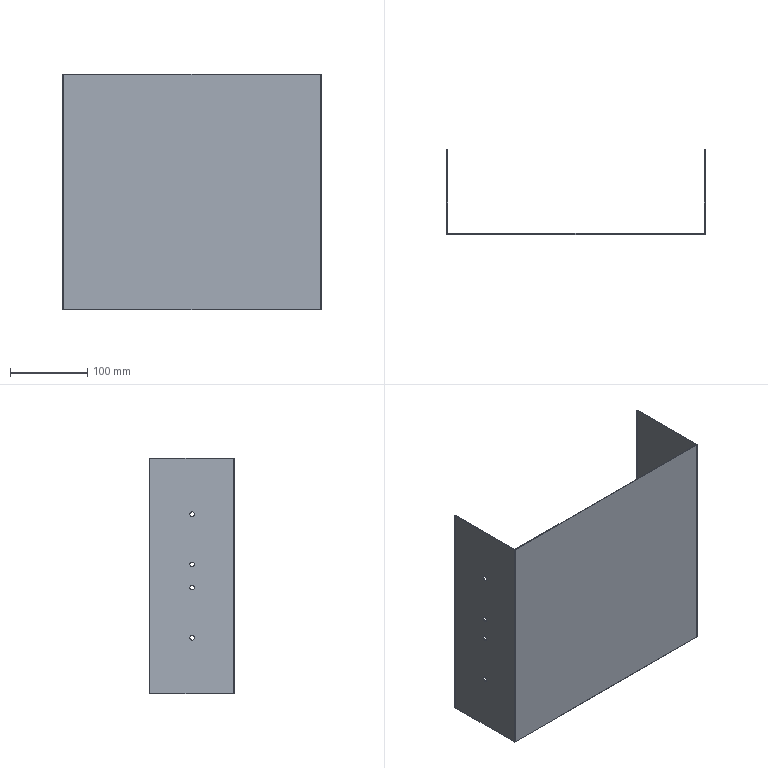Component | SolidWorks | WeldmentDrawing-1_DrawerBox-1 | 1 solid | 38 faces | box 335 x 110 x 305 mm | volume 168282 mm3 | cylinder 20 | plane 18 | commonest cylinder face diameters 6 x16 2.2 x2 0.2 x2
STEP:
#1=COLOUR_RGB('',0.7922,0.8196,0.9333);
#2=FILL_AREA_STYLE_COLOUR('',#1);
#3=FILL_AREA_STYLE('',(#2));
#4=SURFACE_STYLE_FILL_AREA(#3);
#5=SURFACE_SIDE_STYLE('',(#4));
#6=SURFACE_STYLE_USAGE(.BOTH.,#5);
#7=PRESENTATION_STYLE_ASSIGNMENT((#6));
#8=CARTESIAN_POINT('',(-7.849,-9.742,-0.09842));
#9=VERTEX_POINT('',#8);
#10=CARTESIAN_POINT('',(-7.849,-9.506,-0.09842));
#11=VERTEX_POINT('',#10);
#12=CARTESIAN_POINT('',(-7.849,-9.624,-0.09842));
#13=DIRECTION('',(1.,-0.,0.));
#14=DIRECTION('',(0.,-1.,0.));
#15=AXIS2_PLACEMENT_3D('',#12,#13,#14);
#16=CIRCLE('',#15,0.1181);
#17=EDGE_CURVE('',#9,#11,#16,.T.);
#18=ORIENTED_EDGE('',*,*,#17,.F.);
#19=CARTESIAN_POINT('',(-7.809,-9.742,-0.09842));
#20=VERTEX_POINT('',#19);
#21=CARTESIAN_POINT('',(-7.849,-9.742,-0.09842));
#22=DIRECTION('',(1.,-0.,0.));
#23=VECTOR('',#22,39.37);
#24=LINE('',#21,#23);
#25=EDGE_CURVE('',#9,#20,#24,.T.);
#26=ORIENTED_EDGE('',*,*,#25,.T.);
#27=CARTESIAN_POINT('',(-7.809,-9.506,-0.09842));
#28=VERTEX_POINT('',#27);
#29=CARTESIAN_POINT('',(-7.809,-9.624,-0.09842));
#30=DIRECTION('',(1.,0.,0.));
#31=DIRECTION('',(0.,1.,0.));
#32=AXIS2_PLACEMENT_3D('',#29,#30,#31);
#33=CIRCLE('',#32,0.1181);
#34=EDGE_CURVE('',#20,#28,#33,.T.);
#35=ORIENTED_EDGE('',*,*,#34,.T.);
#36=CARTESIAN_POINT('',(-7.849,-9.506,-0.09842));
#37=DIRECTION('',(1.,-0.,0.));
#38=VECTOR('',#37,39.37);
#39=LINE('',#36,#38);
#40=EDGE_CURVE('',#11,#28,#39,.T.);
#41=ORIENTED_EDGE('',*,*,#40,.F.);
#42=EDGE_LOOP('',(#18,#26,#35,#41));
#43=FACE_OUTER_BOUND('',#42,.T.);
#44=CARTESIAN_POINT('',(-7.849,-9.624,-0.09842));
#45=DIRECTION('',(1.,-0.,0.));
#46=DIRECTION('',(0.,1.,0.));
#47=AXIS2_PLACEMENT_3D('',#44,#45,#46);
#48=CYLINDRICAL_SURFACE('',#47,0.1181);
#49=ADVANCED_FACE('',(#43),#48,.F.);
#50=CARTESIAN_POINT('',(5.301,-9.506,-0.09842));
#51=VERTEX_POINT('',#50);
#52=CARTESIAN_POINT('',(5.301,-9.742,-0.09842));
#53=VERTEX_POINT('',#52);
#54=CARTESIAN_POINT('',(5.301,-9.624,-0.09842));
#55=DIRECTION('',(-1.,0.,0.));
#56=DIRECTION('',(0.,-1.,0.));
#57=AXIS2_PLACEMENT_3D('',#54,#55,#56);
#58=CIRCLE('',#57,0.1181);
#59=EDGE_CURVE('',#51,#53,#58,.T.);
#60=ORIENTED_EDGE('',*,*,#59,.T.);
#61=CARTESIAN_POINT('',(5.34,-9.742,-0.09842));
#62=VERTEX_POINT('',#61);
#63=CARTESIAN_POINT('',(-7.849,-9.742,-0.09842));
#64=DIRECTION('',(1.,-0.,0.));
#65=VECTOR('',#64,39.37);
#66=LINE('',#63,#65);
#67=EDGE_CURVE('',#53,#62,#66,.T.);
#68=ORIENTED_EDGE('',*,*,#67,.T.);
#69=CARTESIAN_POINT('',(5.34,-9.506,-0.09842));
#70=VERTEX_POINT('',#69);
#71=CARTESIAN_POINT('',(5.34,-9.624,-0.09842));
#72=DIRECTION('',(1.,-0.,0.));
#73=DIRECTION('',(0.,-1.,0.));
#74=AXIS2_PLACEMENT_3D('',#71,#72,#73);
#75=CIRCLE('',#74,0.1181);
#76=EDGE_CURVE('',#62,#70,#75,.T.);
#77=ORIENTED_EDGE('',*,*,#76,.T.);
#78=CARTESIAN_POINT('',(-7.849,-9.506,-0.09842));
#79=DIRECTION('',(1.,-0.,0.));
#80=VECTOR('',#79,39.37);
#81=LINE('',#78,#80);
#82=EDGE_CURVE('',#51,#70,#81,.T.);
#83=ORIENTED_EDGE('',*,*,#82,.F.);
#84=EDGE_LOOP('',(#60,#68,#77,#83));
#85=FACE_OUTER_BOUND('',#84,.T.);
#86=CARTESIAN_POINT('',(-7.849,-9.624,-0.09842));
#87=DIRECTION('',(1.,-0.,0.));
#88=DIRECTION('',(0.,1.,0.));
#89=AXIS2_PLACEMENT_3D('',#86,#87,#88);
#90=CYLINDRICAL_SURFACE('',#89,0.1181);
#91=ADVANCED_FACE('',(#85),#90,.F.);
#92=CARTESIAN_POINT('',(-7.849,-9.742,2.461));
#93=VERTEX_POINT('',#92);
#94=CARTESIAN_POINT('',(-7.849,-9.506,2.461));
#95=VERTEX_POINT('',#94);
#96=CARTESIAN_POINT('',(-7.849,-9.624,2.461));
#97=DIRECTION('',(1.,-0.,0.));
#98=DIRECTION('',(0.,-1.,0.));
#99=AXIS2_PLACEMENT_3D('',#96,#97,#98);
#100=CIRCLE('',#99,0.1181);
#101=EDGE_CURVE('',#93,#95,#100,.T.);
#102=ORIENTED_EDGE('',*,*,#101,.F.);
#103=CARTESIAN_POINT('',(-7.809,-9.742,2.461));
#104=VERTEX_POINT('',#103);
#105=CARTESIAN_POINT('',(-7.849,-9.742,2.461));
#106=DIRECTION('',(1.,-0.,0.));
#107=VECTOR('',#106,39.37);
#108=LINE('',#105,#107);
#109=EDGE_CURVE('',#93,#104,#108,.T.);
#110=ORIENTED_EDGE('',*,*,#109,.T.);
#111=CARTESIAN_POINT('',(-7.809,-9.506,2.461));
#112=VERTEX_POINT('',#111);
#113=CARTESIAN_POINT('',(-7.809,-9.624,2.461));
#114=DIRECTION('',(1.,0.,0.));
#115=DIRECTION('',(0.,1.,0.));
#116=AXIS2_PLACEMENT_3D('',#113,#114,#115);
#117=CIRCLE('',#116,0.1181);
#118=EDGE_CURVE('',#104,#112,#117,.T.);
#119=ORIENTED_EDGE('',*,*,#118,.T.);
#120=CARTESIAN_POINT('',(-7.849,-9.506,2.461));
#121=DIRECTION('',(1.,-0.,0.));
#122=VECTOR('',#121,39.37);
#123=LINE('',#120,#122);
#124=EDGE_CURVE('',#95,#112,#123,.T.);
#125=ORIENTED_EDGE('',*,*,#124,.F.);
#126=EDGE_LOOP('',(#102,#110,#119,#125));
#127=FACE_OUTER_BOUND('',#126,.T.);
#128=CARTESIAN_POINT('',(-7.849,-9.624,2.461));
#129=DIRECTION('',(1.,-0.,0.));
#130=DIRECTION('',(0.,1.,0.));
#131=AXIS2_PLACEMENT_3D('',#128,#129,#130);
#132=CYLINDRICAL_SURFACE('',#131,0.1181);
#133=ADVANCED_FACE('',(#127),#132,.F.);
#134=CARTESIAN_POINT('',(5.301,-9.506,2.461));
#135=VERTEX_POINT('',#134);
#136=CARTESIAN_POINT('',(5.301,-9.742,2.461));
#137=VERTEX_POINT('',#136);
#138=CARTESIAN_POINT('',(5.301,-9.624,2.461));
#139=DIRECTION('',(-1.,0.,0.));
#140=DIRECTION('',(0.,-1.,0.));
#141=AXIS2_PLACEMENT_3D('',#138,#139,#140);
#142=CIRCLE('',#141,0.1181);
#143=EDGE_CURVE('',#135,#137,#142,.T.);
#144=ORIENTED_EDGE('',*,*,#143,.T.);
#145=CARTESIAN_POINT('',(5.34,-9.742,2.461));
#146=VERTEX_POINT('',#145);
#147=CARTESIAN_POINT('',(-7.849,-9.742,2.461));
#148=DIRECTION('',(1.,-0.,0.));
#149=VECTOR('',#148,39.37);
#150=LINE('',#147,#149);
#151=EDGE_CURVE('',#137,#146,#150,.T.);
#152=ORIENTED_EDGE('',*,*,#151,.T.);
#153=CARTESIAN_POINT('',(5.34,-9.506,2.461));
#154=VERTEX_POINT('',#153);
#155=CARTESIAN_POINT('',(5.34,-9.624,2.461));
#156=DIRECTION('',(1.,-0.,0.));
#157=DIRECTION('',(0.,-1.,0.));
#158=AXIS2_PLACEMENT_3D('',#155,#156,#157);
#159=CIRCLE('',#158,0.1181);
#160=EDGE_CURVE('',#146,#154,#159,.T.);
#161=ORIENTED_EDGE('',*,*,#160,.T.);
#162=CARTESIAN_POINT('',(-7.849,-9.506,2.461));
#163=DIRECTION('',(1.,-0.,0.));
#164=VECTOR('',#163,39.37);
#165=LINE('',#162,#164);
#166=EDGE_CURVE('',#135,#154,#165,.T.);
#167=ORIENTED_EDGE('',*,*,#166,.F.);
#168=EDGE_LOOP('',(#144,#152,#161,#167));
#169=FACE_OUTER_BOUND('',#168,.T.);
#170=CARTESIAN_POINT('',(-7.849,-9.624,2.461));
#171=DIRECTION('',(1.,-0.,0.));
#172=DIRECTION('',(0.,1.,0.));
#173=AXIS2_PLACEMENT_3D('',#170,#171,#172);
#174=CYLINDRICAL_SURFACE('',#173,0.1181);
#175=ADVANCED_FACE('',(#169),#174,.F.);
#176=CARTESIAN_POINT('',(-7.849,-9.742,3.642));
#177=VERTEX_POINT('',#176);
#178=CARTESIAN_POINT('',(-7.849,-9.506,3.642));
#179=VERTEX_POINT('',#178);
#180=CARTESIAN_POINT('',(-7.849,-9.624,3.642));
#181=DIRECTION('',(1.,-0.,0.));
#182=DIRECTION('',(0.,1.,0.));
#183=AXIS2_PLACEMENT_3D('',#180,#181,#182);
#184=CIRCLE('',#183,0.1181);
#185=EDGE_CURVE('',#177,#179,#184,.T.);
#186=ORIENTED_EDGE('',*,*,#185,.F.);
#187=CARTESIAN_POINT('',(-7.809,-9.742,3.642));
#188=VERTEX_POINT('',#187);
#189=CARTESIAN_POINT('',(-7.849,-9.742,3.642));
#190=DIRECTION('',(1.,-0.,0.));
#191=VECTOR('',#190,39.37);
#192=LINE('',#189,#191);
#193=EDGE_CURVE('',#177,#188,#192,.T.);
#194=ORIENTED_EDGE('',*,*,#193,.T.);
#195=CARTESIAN_POINT('',(-7.809,-9.506,3.642));
#196=VERTEX_POINT('',#195);
#197=CARTESIAN_POINT('',(-7.809,-9.624,3.642));
#198=DIRECTION('',(1.,0.,0.));
#199=DIRECTION('',(0.,1.,0.));
#200=AXIS2_PLACEMENT_3D('',#197,#198,#199);
#201=CIRCLE('',#200,0.1181);
#202=EDGE_CURVE('',#188,#196,#201,.T.);
#203=ORIENTED_EDGE('',*,*,#202,.T.);
#204=CARTESIAN_POINT('',(-7.849,-9.506,3.642));
#205=DIRECTION('',(1.,-0.,0.));
#206=VECTOR('',#205,39.37);
#207=LINE('',#204,#206);
#208=EDGE_CURVE('',#179,#196,#207,.T.);
#209=ORIENTED_EDGE('',*,*,#208,.F.);
#210=EDGE_LOOP('',(#186,#194,#203,#209));
#211=FACE_OUTER_BOUND('',#210,.T.);
#212=CARTESIAN_POINT('',(-7.849,-9.624,3.642));
#213=DIRECTION('',(1.,-0.,0.));
#214=DIRECTION('',(0.,1.,0.));
#215=AXIS2_PLACEMENT_3D('',#212,#213,#214);
#216=CYLINDRICAL_SURFACE('',#215,0.1181);
#217=ADVANCED_FACE('',(#211),#216,.F.);
#218=CARTESIAN_POINT('',(5.301,-9.506,3.642));
#219=VERTEX_POINT('',#218);
#220=CARTESIAN_POINT('',(5.301,-9.742,3.642));
#221=VERTEX_POINT('',#220);
#222=CARTESIAN_POINT('',(5.301,-9.624,3.642));
#223=DIRECTION('',(-1.,0.,0.));
#224=DIRECTION('',(0.,-1.,0.));
#225=AXIS2_PLACEMENT_3D('',#222,#223,#224);
#226=CIRCLE('',#225,0.1181);
#227=EDGE_CURVE('',#219,#221,#226,.T.);
#228=ORIENTED_EDGE('',*,*,#227,.T.);
#229=CARTESIAN_POINT('',(5.34,-9.742,3.642));
#230=VERTEX_POINT('',#229);
#231=CARTESIAN_POINT('',(-7.849,-9.742,3.642));
#232=DIRECTION('',(1.,-0.,0.));
#233=VECTOR('',#232,39.37);
#234=LINE('',#231,#233);
#235=EDGE_CURVE('',#221,#230,#234,.T.);
#236=ORIENTED_EDGE('',*,*,#235,.T.);
#237=CARTESIAN_POINT('',(5.34,-9.506,3.642));
#238=VERTEX_POINT('',#237);
#239=CARTESIAN_POINT('',(5.34,-9.624,3.642));
#240=DIRECTION('',(1.,-0.,0.));
#241=DIRECTION('',(0.,1.,0.));
#242=AXIS2_PLACEMENT_3D('',#239,#240,#241);
#243=CIRCLE('',#242,0.1181);
#244=EDGE_CURVE('',#230,#238,#243,.T.);
#245=ORIENTED_EDGE('',*,*,#244,.T.);
#246=CARTESIAN_POINT('',(-7.849,-9.506,3.642));
#247=DIRECTION('',(1.,-0.,0.));
#248=VECTOR('',#247,39.37);
#249=LINE('',#246,#248);
#250=EDGE_CURVE('',#219,#238,#249,.T.);
#251=ORIENTED_EDGE('',*,*,#250,.F.);
#252=EDGE_LOOP('',(#228,#236,#245,#251));
#253=FACE_OUTER_BOUND('',#252,.T.);
#254=CARTESIAN_POINT('',(-7.849,-9.624,3.642));
#255=DIRECTION('',(1.,-0.,0.));
#256=DIRECTION('',(0.,1.,0.));
#257=AXIS2_PLACEMENT_3D('',#254,#255,#256);
#258=CYLINDRICAL_SURFACE('',#257,0.1181);
#259=ADVANCED_FACE('',(#253),#258,.F.);
#260=CARTESIAN_POINT('',(-7.849,-9.742,6.201));
#261=VERTEX_POINT('',#260);
#262=CARTESIAN_POINT('',(-7.849,-9.506,6.201));
#263=VERTEX_POINT('',#262);
#264=CARTESIAN_POINT('',(-7.849,-9.624,6.201));
#265=DIRECTION('',(1.,-0.,0.));
#266=DIRECTION('',(0.,1.,0.));
#267=AXIS2_PLACEMENT_3D('',#264,#265,#266);
#268=CIRCLE('',#267,0.1181);
#269=EDGE_CURVE('',#261,#263,#268,.T.);
#270=ORIENTED_EDGE('',*,*,#269,.F.);
#271=CARTESIAN_POINT('',(-7.809,-9.742,6.201));
#272=VERTEX_POINT('',#271);
#273=CARTESIAN_POINT('',(-7.849,-9.742,6.201));
#274=DIRECTION('',(1.,-0.,0.));
#275=VECTOR('',#274,39.37);
#276=LINE('',#273,#275);
#277=EDGE_CURVE('',#261,#272,#276,.T.);
#278=ORIENTED_EDGE('',*,*,#277,.T.);
#279=CARTESIAN_POINT('',(-7.809,-9.506,6.201));
#280=VERTEX_POINT('',#279);
#281=CARTESIAN_POINT('',(-7.809,-9.624,6.201));
#282=DIRECTION('',(1.,0.,0.));
#283=DIRECTION('',(0.,1.,0.));
#284=AXIS2_PLACEMENT_3D('',#281,#282,#283);
#285=CIRCLE('',#284,0.1181);
#286=EDGE_CURVE('',#272,#280,#285,.T.);
#287=ORIENTED_EDGE('',*,*,#286,.T.);
#288=CARTESIAN_POINT('',(-7.849,-9.506,6.201));
#289=DIRECTION('',(1.,-0.,0.));
#290=VECTOR('',#289,39.37);
#291=LINE('',#288,#290);
#292=EDGE_CURVE('',#263,#280,#291,.T.);
#293=ORIENTED_EDGE('',*,*,#292,.F.);
#294=EDGE_LOOP('',(#270,#278,#287,#293));
#295=FACE_OUTER_BOUND('',#294,.T.);
#296=CARTESIAN_POINT('',(-7.849,-9.624,6.201));
#297=DIRECTION('',(1.,-0.,0.));
#298=DIRECTION('',(0.,1.,0.));
#299=AXIS2_PLACEMENT_3D('',#296,#297,#298);
#300=CYLINDRICAL_SURFACE('',#299,0.1181);
#301=ADVANCED_FACE('',(#295),#300,.F.);
#302=CARTESIAN_POINT('',(5.301,-9.506,6.201));
#303=VERTEX_POINT('',#302);
#304=CARTESIAN_POINT('',(5.301,-9.742,6.201));
#305=VERTEX_POINT('',#304);
#306=CARTESIAN_POINT('',(5.301,-9.624,6.201));
#307=DIRECTION('',(-1.,0.,0.));
#308=DIRECTION('',(0.,-1.,0.));
#309=AXIS2_PLACEMENT_3D('',#306,#307,#308);
#310=CIRCLE('',#309,0.1181);
#311=EDGE_CURVE('',#303,#305,#310,.T.);
#312=ORIENTED_EDGE('',*,*,#311,.T.);
#313=CARTESIAN_POINT('',(5.34,-9.742,6.201));
#314=VERTEX_POINT('',#313);
#315=CARTESIAN_POINT('',(-7.849,-9.742,6.201));
#316=DIRECTION('',(1.,-0.,0.));
#317=VECTOR('',#316,39.37);
#318=LINE('',#315,#317);
#319=EDGE_CURVE('',#305,#314,#318,.T.);
#320=ORIENTED_EDGE('',*,*,#319,.T.);
#321=CARTESIAN_POINT('',(5.34,-9.506,6.201));
#322=VERTEX_POINT('',#321);
#323=CARTESIAN_POINT('',(5.34,-9.624,6.201));
#324=DIRECTION('',(1.,-0.,0.));
#325=DIRECTION('',(0.,1.,0.));
#326=AXIS2_PLACEMENT_3D('',#323,#324,#325);
#327=CIRCLE('',#326,0.1181);
#328=EDGE_CURVE('',#314,#322,#327,.T.);
#329=ORIENTED_EDGE('',*,*,#328,.T.);
#330=CARTESIAN_POINT('',(-7.849,-9.506,6.201));
#331=DIRECTION('',(1.,-0.,0.));
#332=VECTOR('',#331,39.37);
#333=LINE('',#330,#332);
#334=EDGE_CURVE('',#303,#322,#333,.T.);
#335=ORIENTED_EDGE('',*,*,#334,.F.);
#336=EDGE_LOOP('',(#312,#320,#329,#335));
#337=FACE_OUTER_BOUND('',#336,.T.);
#338=CARTESIAN_POINT('',(-7.849,-9.624,6.201));
#339=DIRECTION('',(1.,-0.,0.));
#340=DIRECTION('',(0.,1.,0.));
#341=AXIS2_PLACEMENT_3D('',#338,#339,#340);
#342=CYLINDRICAL_SURFACE('',#341,0.1181);
#343=ADVANCED_FACE('',(#337),#342,.F.);
#344=CARTESIAN_POINT('',(5.297,-11.778,-2.953));
#345=VERTEX_POINT('',#344);
#346=CARTESIAN_POINT('',(-7.806,-11.778,-2.953));
#347=VERTEX_POINT('',#346);
#348=CARTESIAN_POINT('',(-7.849,-11.778,-2.953));
#349=DIRECTION('',(-1.,0.,0.));
#350=VECTOR('',#349,39.37);
#351=LINE('',#348,#350);
#352=EDGE_CURVE('',#345,#347,#351,.T.);
#353=ORIENTED_EDGE('',*,*,#352,.F.);
#354=CARTESIAN_POINT('',(5.297,-11.778,9.055));
#355=VERTEX_POINT('',#354);
#356=CARTESIAN_POINT('',(5.297,-11.778,-2.953));
#357=DIRECTION('',(0.,0.,1.));
#358=VECTOR('',#357,39.37);
#359=LINE('',#356,#358);
#360=EDGE_CURVE('',#345,#355,#359,.T.);
#361=ORIENTED_EDGE('',*,*,#360,.T.);
#362=CARTESIAN_POINT('',(-7.806,-11.778,9.055));
#363=VERTEX_POINT('',#362);
#364=CARTESIAN_POINT('',(-7.849,-11.778,9.055));
#365=DIRECTION('',(1.,0.,0.));
#366=VECTOR('',#365,39.37);
#367=LINE('',#364,#366);
#368=EDGE_CURVE('',#363,#355,#367,.T.);
#369=ORIENTED_EDGE('',*,*,#368,.F.);
#370=CARTESIAN_POINT('',(-7.806,-11.778,9.055));
#371=DIRECTION('',(0.,0.,-1.));
#372=VECTOR('',#371,39.37);
#373=LINE('',#370,#372);
#374=EDGE_CURVE('',#363,#347,#373,.T.);
#375=ORIENTED_EDGE('',*,*,#374,.T.);
#376=EDGE_LOOP('',(#353,#361,#369,#375));
#377=FACE_OUTER_BOUND('',#376,.T.);
#378=CARTESIAN_POINT('',(-5.646,-11.778,6.989));
#379=DIRECTION('',(0.,-1.,0.));
#380=DIRECTION('',(0.,0.,-1.));
#381=AXIS2_PLACEMENT_3D('',#378,#379,#380);
#382=PLANE('',#381);
#383=ADVANCED_FACE('',(#377),#382,.T.);
#384=CARTESIAN_POINT('',(5.297,-11.738,-2.953));
#385=VERTEX_POINT('',#384);
#386=CARTESIAN_POINT('',(5.297,-11.738,9.055));
#387=VERTEX_POINT('',#386);
#388=CARTESIAN_POINT('',(5.297,-11.738,-2.953));
#389=DIRECTION('',(0.,0.,1.));
#390=VECTOR('',#389,39.37);
#391=LINE('',#388,#390);
#392=EDGE_CURVE('',#385,#387,#391,.T.);
#393=ORIENTED_EDGE('',*,*,#392,.F.);
#394=CARTESIAN_POINT('',(-7.806,-11.738,-2.953));
#395=VERTEX_POINT('',#394);
#396=CARTESIAN_POINT('',(-7.849,-11.738,-2.953));
#397=DIRECTION('',(-1.,0.,0.));
#398=VECTOR('',#397,39.37);
#399=LINE('',#396,#398);
#400=EDGE_CURVE('',#385,#395,#399,.T.);
#401=ORIENTED_EDGE('',*,*,#400,.T.);
#402=CARTESIAN_POINT('',(-7.806,-11.738,9.055));
#403=VERTEX_POINT('',#402);
#404=CARTESIAN_POINT('',(-7.806,-11.738,9.055));
#405=DIRECTION('',(0.,0.,-1.));
#406=VECTOR('',#405,39.37);
#407=LINE('',#404,#406);
#408=EDGE_CURVE('',#403,#395,#407,.T.);
#409=ORIENTED_EDGE('',*,*,#408,.F.);
#410=CARTESIAN_POINT('',(-7.849,-11.738,9.055));
#411=DIRECTION('',(1.,0.,0.));
#412=VECTOR('',#411,39.37);
#413=LINE('',#410,#412);
#414=EDGE_CURVE('',#403,#387,#413,.T.);
#415=ORIENTED_EDGE('',*,*,#414,.T.);
#416=EDGE_LOOP('',(#393,#401,#409,#415));
#417=FACE_OUTER_BOUND('',#416,.T.);
#418=CARTESIAN_POINT('',(-5.646,-11.738,6.989));
#419=DIRECTION('',(0.,-1.,0.));
#420=DIRECTION('',(0.,0.,-1.));
#421=AXIS2_PLACEMENT_3D('',#418,#419,#420);
#422=PLANE('',#421);
#423=ADVANCED_FACE('',(#417),#422,.F.);
#424=ORIENTED_EDGE('',*,*,#400,.F.);
#425=CARTESIAN_POINT('',(5.297,-11.738,-2.953));
#426=DIRECTION('',(0.,-1.,-0.));
#427=VECTOR('',#426,39.37);
#428=LINE('',#425,#427);
#429=EDGE_CURVE('',#385,#345,#428,.T.);
#430=ORIENTED_EDGE('',*,*,#429,.T.);
#431=ORIENTED_EDGE('',*,*,#352,.T.);
#432=CARTESIAN_POINT('',(-7.806,-11.738,-2.953));
#433=DIRECTION('',(0.,-1.,0.));
#434=VECTOR('',#433,39.37);
#435=LINE('',#432,#434);
#436=EDGE_CURVE('',#395,#347,#435,.T.);
#437=ORIENTED_EDGE('',*,*,#436,.F.);
#438=EDGE_LOOP('',(#424,#430,#431,#437));
#439=FACE_OUTER_BOUND('',#438,.T.);
#440=CARTESIAN_POINT('',(-7.849,-11.778,-2.953));
#441=DIRECTION('',(0.,0.,-1.));
#442=DIRECTION('',(-1.,0.,0.));
#443=AXIS2_PLACEMENT_3D('',#440,#441,#442);
#444=PLANE('',#443);
#445=ADVANCED_FACE('',(#439),#444,.T.);
#446=CARTESIAN_POINT('',(5.297,-11.738,9.055));
#447=DIRECTION('',(0.,-1.,0.));
#448=VECTOR('',#447,39.37);
#449=LINE('',#446,#448);
#450=EDGE_CURVE('',#387,#355,#449,.T.);
#451=ORIENTED_EDGE('',*,*,#450,.F.);
#452=ORIENTED_EDGE('',*,*,#414,.F.);
#453=CARTESIAN_POINT('',(-7.806,-11.738,9.055));
#454=DIRECTION('',(0.,-1.,-0.));
#455=VECTOR('',#454,39.37);
#456=LINE('',#453,#455);
#457=EDGE_CURVE('',#403,#363,#456,.T.);
#458=ORIENTED_EDGE('',*,*,#457,.T.);
#459=ORIENTED_EDGE('',*,*,#368,.T.);
#460=EDGE_LOOP('',(#451,#452,#458,#459));
#461=FACE_OUTER_BOUND('',#460,.T.);
#462=CARTESIAN_POINT('',(-7.849,-11.778,9.055));
#463=DIRECTION('',(0.,0.,1.));
#464=DIRECTION('',(1.,0.,0.));
#465=AXIS2_PLACEMENT_3D('',#462,#463,#464);
#466=PLANE('',#465);
#467=ADVANCED_FACE('',(#461),#466,.T.);
#468=CARTESIAN_POINT('',(-7.809,-11.734,-2.953));
#469=VERTEX_POINT('',#468);
#470=CARTESIAN_POINT('',(-7.849,-11.734,-2.953));
#471=VERTEX_POINT('',#470);
#472=CARTESIAN_POINT('',(-7.849,-11.734,-2.953));
#473=DIRECTION('',(-1.,-0.,0.));
#474=VECTOR('',#473,39.37);
#475=LINE('',#472,#474);
#476=EDGE_CURVE('',#469,#471,#475,.T.);
#477=ORIENTED_EDGE('',*,*,#476,.F.);
#478=CARTESIAN_POINT('',(-7.806,-11.734,-2.953));
#479=DIRECTION('',(0.,0.,-1.));
#480=DIRECTION('',(0.,-1.,0.));
#481=AXIS2_PLACEMENT_3D('',#478,#479,#480);
#482=CIRCLE('',#481,0.003937);
#483=EDGE_CURVE('',#395,#469,#482,.T.);
#484=ORIENTED_EDGE('',*,*,#483,.F.);
#485=ORIENTED_EDGE('',*,*,#436,.T.);
#486=CARTESIAN_POINT('',(-7.806,-11.734,-2.953));
#487=DIRECTION('',(0.,0.,-1.));
#488=DIRECTION('',(0.,-1.,0.));
#489=AXIS2_PLACEMENT_3D('',#486,#487,#488);
#490=CIRCLE('',#489,0.04331);
#491=EDGE_CURVE('',#347,#471,#490,.T.);
#492=ORIENTED_EDGE('',*,*,#491,.T.);
#493=EDGE_LOOP('',(#477,#484,#485,#492));
#494=FACE_OUTER_BOUND('',#493,.T.);
#495=CARTESIAN_POINT('',(-7.806,-11.734,-2.953));
#496=DIRECTION('',(0.,0.,-1.));
#497=DIRECTION('',(0.,1.,0.));
#498=AXIS2_PLACEMENT_3D('',#495,#496,#497);
#499=PLANE('',#498);
#500=ADVANCED_FACE('',(#494),#499,.T.);
#501=CARTESIAN_POINT('',(-7.809,-11.734,9.055));
#502=VERTEX_POINT('',#501);
#503=CARTESIAN_POINT('',(-7.806,-11.734,9.055));
#504=DIRECTION('',(0.,-0.,1.));
#505=DIRECTION('',(0.,-1.,0.));
#506=AXIS2_PLACEMENT_3D('',#503,#504,#505);
#507=CIRCLE('',#506,0.003937);
#508=EDGE_CURVE('',#502,#403,#507,.T.);
#509=ORIENTED_EDGE('',*,*,#508,.F.);
#510=CARTESIAN_POINT('',(-7.849,-11.734,9.055));
#511=VERTEX_POINT('',#510);
#512=CARTESIAN_POINT('',(-7.809,-11.734,9.055));
#513=DIRECTION('',(-1.,-0.,0.));
#514=VECTOR('',#513,39.37);
#515=LINE('',#512,#514);
#516=EDGE_CURVE('',#502,#511,#515,.T.);
#517=ORIENTED_EDGE('',*,*,#516,.T.);
#518=CARTESIAN_POINT('',(-7.806,-11.734,9.055));
#519=DIRECTION('',(0.,-0.,1.));
#520=DIRECTION('',(0.,-1.,0.));
#521=AXIS2_PLACEMENT_3D('',#518,#519,#520);
#522=CIRCLE('',#521,0.04331);
#523=EDGE_CURVE('',#511,#363,#522,.T.);
#524=ORIENTED_EDGE('',*,*,#523,.T.);
#525=ORIENTED_EDGE('',*,*,#457,.F.);
#526=EDGE_LOOP('',(#509,#517,#524,#525));
#527=FACE_OUTER_BOUND('',#526,.T.);
#528=CARTESIAN_POINT('',(-7.806,-11.734,9.055));
#529=DIRECTION('',(0.,0.,-1.));
#530=DIRECTION('',(0.,1.,0.));
#531=AXIS2_PLACEMENT_3D('',#528,#529,#530);
#532=PLANE('',#531);
#533=ADVANCED_FACE('',(#527),#532,.F.);
#534=ORIENTED_EDGE('',*,*,#374,.F.);
#535=ORIENTED_EDGE('',*,*,#523,.F.);
#536=CARTESIAN_POINT('',(-7.849,-11.734,-2.953));
#537=DIRECTION('',(-0.,0.,-1.));
#538=VECTOR('',#537,39.37);
#539=LINE('',#536,#538);
#540=EDGE_CURVE('',#511,#471,#539,.T.);
#541=ORIENTED_EDGE('',*,*,#540,.T.);
#542=ORIENTED_EDGE('',*,*,#491,.F.);
#543=EDGE_LOOP('',(#534,#535,#541,#542));
#544=FACE_OUTER_BOUND('',#543,.T.);
#545=CARTESIAN_POINT('',(-7.806,-11.734,9.055));
#546=DIRECTION('',(0.,-0.,1.));
#547=DIRECTION('',(-1.,0.,0.));
#548=AXIS2_PLACEMENT_3D('',#545,#546,#547);
#549=CYLINDRICAL_SURFACE('',#548,0.04331);
#550=ADVANCED_FACE('',(#544),#549,.T.);
#551=ORIENTED_EDGE('',*,*,#408,.T.);
#552=ORIENTED_EDGE('',*,*,#483,.T.);
#553=CARTESIAN_POINT('',(-7.809,-11.734,-2.953));
#554=DIRECTION('',(0.,-0.,1.));
#555=VECTOR('',#554,39.37);
#556=LINE('',#553,#555);
#557=EDGE_CURVE('',#469,#502,#556,.T.);
#558=ORIENTED_EDGE('',*,*,#557,.T.);
#559=ORIENTED_EDGE('',*,*,#508,.T.);
#560=EDGE_LOOP('',(#551,#552,#558,#559));
#561=FACE_OUTER_BOUND('',#560,.T.);
#562=CARTESIAN_POINT('',(-7.806,-11.734,9.055));
#563=DIRECTION('',(0.,-0.,1.));
#564=DIRECTION('',(-1.,0.,0.));
#565=AXIS2_PLACEMENT_3D('',#562,#563,#564);
#566=CYLINDRICAL_SURFACE('',#565,0.003937);
#567=ADVANCED_FACE('',(#561),#566,.F.);
#568=ORIENTED_EDGE('',*,*,#476,.T.);
#569=CARTESIAN_POINT('',(-7.849,-7.447,-2.953));
#570=VERTEX_POINT('',#569);
#571=CARTESIAN_POINT('',(-7.849,-11.738,-2.953));
#572=DIRECTION('',(0.,-1.,0.));
#573=VECTOR('',#572,39.37);
#574=LINE('',#571,#573);
#575=EDGE_CURVE('',#570,#471,#574,.T.);
#576=ORIENTED_EDGE('',*,*,#575,.F.);
#577=CARTESIAN_POINT('',(-7.809,-7.447,-2.953));
#578=VERTEX_POINT('',#577);
#579=CARTESIAN_POINT('',(-7.849,-7.447,-2.953));
#580=DIRECTION('',(1.,0.,0.));
#581=VECTOR('',#580,39.37);
#582=LINE('',#579,#581);
#583=EDGE_CURVE('',#570,#578,#582,.T.);
#584=ORIENTED_EDGE('',*,*,#583,.T.);
#585=CARTESIAN_POINT('',(-7.809,-11.738,-2.953));
#586=DIRECTION('',(0.,-1.,0.));
#587=VECTOR('',#586,39.37);
#588=LINE('',#585,#587);
#589=EDGE_CURVE('',#578,#469,#588,.T.);
#590=ORIENTED_EDGE('',*,*,#589,.T.);
#591=EDGE_LOOP('',(#568,#576,#584,#590));
#592=FACE_OUTER_BOUND('',#591,.T.);
#593=CARTESIAN_POINT('',(-7.849,-11.738,-2.953));
#594=DIRECTION('',(0.,0.,1.));
#595=DIRECTION('',(1.,0.,0.));
#596=AXIS2_PLACEMENT_3D('',#593,#594,#595);
#597=PLANE('',#596);
#598=ADVANCED_FACE('',(#592),#597,.F.);
#599=ORIENTED_EDGE('',*,*,#516,.F.);
#600=CARTESIAN_POINT('',(-7.809,-7.447,9.055));
#601=VERTEX_POINT('',#600);
#602=CARTESIAN_POINT('',(-7.809,-7.447,9.055));
#603=DIRECTION('',(-0.,1.,0.));
#604=VECTOR('',#603,39.37);
#605=LINE('',#602,#604);
#606=EDGE_CURVE('',#502,#601,#605,.T.);
#607=ORIENTED_EDGE('',*,*,#606,.T.);
#608=CARTESIAN_POINT('',(-7.849,-7.447,9.055));
#609=VERTEX_POINT('',#608);
#610=CARTESIAN_POINT('',(-7.849,-7.447,9.055));
#611=DIRECTION('',(1.,0.,0.));
#612=VECTOR('',#611,39.37);
#613=LINE('',#610,#612);
#614=EDGE_CURVE('',#609,#601,#613,.T.);
#615=ORIENTED_EDGE('',*,*,#614,.F.);
#616=CARTESIAN_POINT('',(-7.849,-11.738,9.055));
#617=DIRECTION('',(-0.,1.,0.));
#618=VECTOR('',#617,39.37);
#619=LINE('',#616,#618);
#620=EDGE_CURVE('',#511,#609,#619,.T.);
#621=ORIENTED_EDGE('',*,*,#620,.F.);
#622=EDGE_LOOP('',(#599,#607,#615,#621));
#623=FACE_OUTER_BOUND('',#622,.T.);
#624=CARTESIAN_POINT('',(-7.849,-7.447,9.055));
#625=DIRECTION('',(0.,0.,-1.));
#626=DIRECTION('',(-1.,0.,0.));
#627=AXIS2_PLACEMENT_3D('',#624,#625,#626);
#628=PLANE('',#627);
#629=ADVANCED_FACE('',(#623),#628,.F.);
#630=CARTESIAN_POINT('',(-7.849,-9.624,-0.09842));
#631=DIRECTION('',(1.,-0.,0.));
#632=DIRECTION('',(0.,-1.,0.));
#633=AXIS2_PLACEMENT_3D('',#630,#631,#632);
#634=CIRCLE('',#633,0.1181);
#635=EDGE_CURVE('',#11,#9,#634,.T.);
#636=ORIENTED_EDGE('',*,*,#635,.T.);
#637=ORIENTED_EDGE('',*,*,#17,.T.);
#638=EDGE_LOOP('',(#636,#637));
#639=FACE_BOUND('',#638,.T.);
#640=CARTESIAN_POINT('',(-7.849,-9.624,2.461));
#641=DIRECTION('',(1.,-0.,0.));
#642=DIRECTION('',(0.,-1.,0.));
#643=AXIS2_PLACEMENT_3D('',#640,#641,#642);
#644=CIRCLE('',#643,0.1181);
#645=EDGE_CURVE('',#95,#93,#644,.T.);
#646=ORIENTED_EDGE('',*,*,#645,.T.);
#647=ORIENTED_EDGE('',*,*,#101,.T.);
#648=EDGE_LOOP('',(#646,#647));
#649=FACE_BOUND('',#648,.T.);
#650=CARTESIAN_POINT('',(-7.849,-9.624,3.642));
#651=DIRECTION('',(1.,-0.,0.));
#652=DIRECTION('',(0.,1.,0.));
#653=AXIS2_PLACEMENT_3D('',#650,#651,#652);
#654=CIRCLE('',#653,0.1181);
#655=EDGE_CURVE('',#179,#177,#654,.T.);
#656=ORIENTED_EDGE('',*,*,#655,.T.);
#657=ORIENTED_EDGE('',*,*,#185,.T.);
#658=EDGE_LOOP('',(#656,#657));
#659=FACE_BOUND('',#658,.T.);
#660=CARTESIAN_POINT('',(-7.849,-9.624,6.201));
#661=DIRECTION('',(1.,-0.,0.));
#662=DIRECTION('',(0.,1.,0.));
#663=AXIS2_PLACEMENT_3D('',#660,#661,#662);
#664=CIRCLE('',#663,0.1181);
#665=EDGE_CURVE('',#263,#261,#664,.T.);
#666=ORIENTED_EDGE('',*,*,#665,.T.);
#667=ORIENTED_EDGE('',*,*,#269,.T.);
#668=EDGE_LOOP('',(#666,#667));
#669=FACE_BOUND('',#668,.T.);
#670=ORIENTED_EDGE('',*,*,#540,.F.);
#671=ORIENTED_EDGE('',*,*,#620,.T.);
#672=CARTESIAN_POINT('',(-7.849,-7.447,6.989));
#673=DIRECTION('',(0.,0.,-1.));
#674=VECTOR('',#673,39.37);
#675=LINE('',#672,#674);
#676=EDGE_CURVE('',#609,#570,#675,.T.);
#677=ORIENTED_EDGE('',*,*,#676,.T.);
#678=ORIENTED_EDGE('',*,*,#575,.T.);
#679=EDGE_LOOP('',(#670,#671,#677,#678));
#680=FACE_OUTER_BOUND('',#679,.T.);
#681=CARTESIAN_POINT('',(-7.849,-11.738,6.989));
#682=DIRECTION('',(1.,0.,0.));
#683=DIRECTION('',(-0.,1.,0.));
#684=AXIS2_PLACEMENT_3D('',#681,#682,#683);
#685=PLANE('',#684);
#686=ADVANCED_FACE('',(#639,#649,#659,#669,#680),#685,.F.);
#687=CARTESIAN_POINT('',(-7.809,-9.624,-0.09842));
#688=DIRECTION('',(1.,0.,0.));
#689=DIRECTION('',(0.,1.,0.));
#690=AXIS2_PLACEMENT_3D('',#687,#688,#689);
#691=CIRCLE('',#690,0.1181);
#692=EDGE_CURVE('',#28,#20,#691,.T.);
#693=ORIENTED_EDGE('',*,*,#692,.F.);
#694=ORIENTED_EDGE('',*,*,#34,.F.);
#695=EDGE_LOOP('',(#693,#694));
#696=FACE_BOUND('',#695,.T.);
#697=CARTESIAN_POINT('',(-7.809,-9.624,2.461));
#698=DIRECTION('',(1.,0.,0.));
#699=DIRECTION('',(0.,1.,0.));
#700=AXIS2_PLACEMENT_3D('',#697,#698,#699);
#701=CIRCLE('',#700,0.1181);
#702=EDGE_CURVE('',#112,#104,#701,.T.);
#703=ORIENTED_EDGE('',*,*,#702,.F.);
#704=ORIENTED_EDGE('',*,*,#118,.F.);
#705=EDGE_LOOP('',(#703,#704));
#706=FACE_BOUND('',#705,.T.);
#707=CARTESIAN_POINT('',(-7.809,-9.624,3.642));
#708=DIRECTION('',(1.,0.,0.));
#709=DIRECTION('',(0.,1.,0.));
#710=AXIS2_PLACEMENT_3D('',#707,#708,#709);
#711=CIRCLE('',#710,0.1181);
#712=EDGE_CURVE('',#196,#188,#711,.T.);
#713=ORIENTED_EDGE('',*,*,#712,.F.);
#714=ORIENTED_EDGE('',*,*,#202,.F.);
#715=EDGE_LOOP('',(#713,#714));
#716=FACE_BOUND('',#715,.T.);
#717=CARTESIAN_POINT('',(-7.809,-9.624,6.201));
#718=DIRECTION('',(1.,0.,0.));
#719=DIRECTION('',(0.,1.,0.));
#720=AXIS2_PLACEMENT_3D('',#717,#718,#719);
#721=CIRCLE('',#720,0.1181);
#722=EDGE_CURVE('',#280,#272,#721,.T.);
#723=ORIENTED_EDGE('',*,*,#722,.F.);
#724=ORIENTED_EDGE('',*,*,#286,.F.);
#725=EDGE_LOOP('',(#723,#724));
#726=FACE_BOUND('',#725,.T.);
#727=ORIENTED_EDGE('',*,*,#606,.F.);
#728=ORIENTED_EDGE('',*,*,#557,.F.);
#729=ORIENTED_EDGE('',*,*,#589,.F.);
#730=CARTESIAN_POINT('',(-7.809,-7.447,-2.953));
#731=DIRECTION('',(0.,0.,-1.));
#732=VECTOR('',#731,39.37);
#733=LINE('',#730,#732);
#734=EDGE_CURVE('',#601,#578,#733,.T.);
#735=ORIENTED_EDGE('',*,*,#734,.F.);
#736=EDGE_LOOP('',(#727,#728,#729,#735));
#737=FACE_OUTER_BOUND('',#736,.T.);
#738=CARTESIAN_POINT('',(-7.809,-11.738,6.989));
#739=DIRECTION('',(1.,0.,0.));
#740=DIRECTION('',(-0.,1.,0.));
#741=AXIS2_PLACEMENT_3D('',#738,#739,#740);
#742=PLANE('',#741);
#743=ADVANCED_FACE('',(#696,#706,#716,#726,#737),#742,.T.);
#744=ORIENTED_EDGE('',*,*,#734,.T.);
#745=ORIENTED_EDGE('',*,*,#583,.F.);
#746=ORIENTED_EDGE('',*,*,#676,.F.);
#747=ORIENTED_EDGE('',*,*,#614,.T.);
#748=EDGE_LOOP('',(#744,#745,#746,#747));
#749=FACE_OUTER_BOUND('',#748,.T.);
#750=CARTESIAN_POINT('',(-7.849,-7.447,-2.953));
#751=DIRECTION('',(0.,-1.,0.));
#752=DIRECTION('',(1.,0.,0.));
#753=AXIS2_PLACEMENT_3D('',#750,#751,#752);
#754=PLANE('',#753);
#755=ADVANCED_FACE('',(#749),#754,.F.);
#756=CARTESIAN_POINT('',(5.301,-11.734,9.055));
#757=VERTEX_POINT('',#756);
#758=CARTESIAN_POINT('',(5.34,-11.734,9.055));
#759=VERTEX_POINT('',#758);
#760=CARTESIAN_POINT('',(5.34,-11.734,9.055));
#761=DIRECTION('',(1.,-0.,0.));
#762=VECTOR('',#761,39.37);
#763=LINE('',#760,#762);
#764=EDGE_CURVE('',#757,#759,#763,.T.);
#765=ORIENTED_EDGE('',*,*,#764,.F.);
#766=CARTESIAN_POINT('',(5.297,-11.734,9.055));
#767=DIRECTION('',(0.,0.,1.));
#768=DIRECTION('',(-1.,0.,0.));
#769=AXIS2_PLACEMENT_3D('',#766,#767,#768);
#770=CIRCLE('',#769,0.003937);
#771=EDGE_CURVE('',#387,#757,#770,.T.);
#772=ORIENTED_EDGE('',*,*,#771,.F.);
#773=ORIENTED_EDGE('',*,*,#450,.T.);
#774=CARTESIAN_POINT('',(5.297,-11.734,9.055));
#775=DIRECTION('',(0.,0.,1.));
#776=DIRECTION('',(-1.,0.,0.));
#777=AXIS2_PLACEMENT_3D('',#774,#775,#776);
#778=CIRCLE('',#777,0.04331);
#779=EDGE_CURVE('',#355,#759,#778,.T.);
#780=ORIENTED_EDGE('',*,*,#779,.T.);
#781=EDGE_LOOP('',(#765,#772,#773,#780));
#782=FACE_OUTER_BOUND('',#781,.T.);
#783=CARTESIAN_POINT('',(5.297,-11.734,9.055));
#784=DIRECTION('',(0.,0.,1.));
#785=DIRECTION('',(1.,0.,0.));
#786=AXIS2_PLACEMENT_3D('',#783,#784,#785);
#787=PLANE('',#786);
#788=ADVANCED_FACE('',(#782),#787,.T.);
#789=CARTESIAN_POINT('',(5.301,-11.734,-2.953));
#790=VERTEX_POINT('',#789);
#791=CARTESIAN_POINT('',(5.297,-11.734,-2.953));
#792=DIRECTION('',(0.,0.,-1.));
#793=DIRECTION('',(-1.,0.,0.));
#794=AXIS2_PLACEMENT_3D('',#791,#792,#793);
#795=CIRCLE('',#794,0.003937);
#796=EDGE_CURVE('',#790,#385,#795,.T.);
#797=ORIENTED_EDGE('',*,*,#796,.F.);
#798=CARTESIAN_POINT('',(5.34,-11.734,-2.953));
#799=VERTEX_POINT('',#798);
#800=CARTESIAN_POINT('',(5.301,-11.734,-2.953));
#801=DIRECTION('',(1.,-0.,0.));
#802=VECTOR('',#801,39.37);
#803=LINE('',#800,#802);
#804=EDGE_CURVE('',#790,#799,#803,.T.);
#805=ORIENTED_EDGE('',*,*,#804,.T.);
#806=CARTESIAN_POINT('',(5.297,-11.734,-2.953));
#807=DIRECTION('',(0.,0.,-1.));
#808=DIRECTION('',(-1.,0.,0.));
#809=AXIS2_PLACEMENT_3D('',#806,#807,#808);
#810=CIRCLE('',#809,0.04331);
#811=EDGE_CURVE('',#799,#345,#810,.T.);
#812=ORIENTED_EDGE('',*,*,#811,.T.);
#813=ORIENTED_EDGE('',*,*,#429,.F.);
#814=EDGE_LOOP('',(#797,#805,#812,#813));
#815=FACE_OUTER_BOUND('',#814,.T.);
#816=CARTESIAN_POINT('',(5.297,-11.734,-2.953));
#817=DIRECTION('',(0.,0.,1.));
#818=DIRECTION('',(1.,0.,0.));
#819=AXIS2_PLACEMENT_3D('',#816,#817,#818);
#820=PLANE('',#819);
#821=ADVANCED_FACE('',(#815),#820,.F.);
#822=ORIENTED_EDGE('',*,*,#360,.F.);
#823=ORIENTED_EDGE('',*,*,#811,.F.);
#824=CARTESIAN_POINT('',(5.34,-11.734,9.055));
#825=DIRECTION('',(0.,0.,1.));
#826=VECTOR('',#825,39.37);
#827=LINE('',#824,#826);
#828=EDGE_CURVE('',#799,#759,#827,.T.);
#829=ORIENTED_EDGE('',*,*,#828,.T.);
#830=ORIENTED_EDGE('',*,*,#779,.F.);
#831=EDGE_LOOP('',(#822,#823,#829,#830));
#832=FACE_OUTER_BOUND('',#831,.T.);
#833=CARTESIAN_POINT('',(5.297,-11.734,-2.953));
#834=DIRECTION('',(0.,0.,-1.));
#835=DIRECTION('',(1.,0.,0.));
#836=AXIS2_PLACEMENT_3D('',#833,#834,#835);
#837=CYLINDRICAL_SURFACE('',#836,0.04331);
#838=ADVANCED_FACE('',(#832),#837,.T.);
#839=ORIENTED_EDGE('',*,*,#392,.T.);
#840=ORIENTED_EDGE('',*,*,#771,.T.);
#841=CARTESIAN_POINT('',(5.301,-11.734,9.055));
#842=DIRECTION('',(0.,0.,-1.));
#843=VECTOR('',#842,39.37);
#844=LINE('',#841,#843);
#845=EDGE_CURVE('',#757,#790,#844,.T.);
#846=ORIENTED_EDGE('',*,*,#845,.T.);
#847=ORIENTED_EDGE('',*,*,#796,.T.);
#848=EDGE_LOOP('',(#839,#840,#846,#847));
#849=FACE_OUTER_BOUND('',#848,.T.);
#850=CARTESIAN_POINT('',(5.297,-11.734,-2.953));
#851=DIRECTION('',(0.,0.,-1.));
#852=DIRECTION('',(1.,0.,0.));
#853=AXIS2_PLACEMENT_3D('',#850,#851,#852);
#854=CYLINDRICAL_SURFACE('',#853,0.003937);
#855=ADVANCED_FACE('',(#849),#854,.F.);
#856=ORIENTED_EDGE('',*,*,#764,.T.);
#857=CARTESIAN_POINT('',(5.34,-7.447,9.055));
#858=VERTEX_POINT('',#857);
#859=CARTESIAN_POINT('',(5.34,-11.738,9.055));
#860=DIRECTION('',(-0.,-1.,0.));
#861=VECTOR('',#860,39.37);
#862=LINE('',#859,#861);
#863=EDGE_CURVE('',#858,#759,#862,.T.);
#864=ORIENTED_EDGE('',*,*,#863,.F.);
#865=CARTESIAN_POINT('',(5.301,-7.447,9.055));
#866=VERTEX_POINT('',#865);
#867=CARTESIAN_POINT('',(5.34,-7.447,9.055));
#868=DIRECTION('',(-1.,0.,0.));
#869=VECTOR('',#868,39.37);
#870=LINE('',#867,#869);
#871=EDGE_CURVE('',#858,#866,#870,.T.);
#872=ORIENTED_EDGE('',*,*,#871,.T.);
#873=CARTESIAN_POINT('',(5.301,-11.738,9.055));
#874=DIRECTION('',(-0.,-1.,0.));
#875=VECTOR('',#874,39.37);
#876=LINE('',#873,#875);
#877=EDGE_CURVE('',#866,#757,#876,.T.);
#878=ORIENTED_EDGE('',*,*,#877,.T.);
#879=EDGE_LOOP('',(#856,#864,#872,#878));
#880=FACE_OUTER_BOUND('',#879,.T.);
#881=CARTESIAN_POINT('',(5.34,-11.738,9.055));
#882=DIRECTION('',(0.,0.,-1.));
#883=DIRECTION('',(-1.,0.,0.));
#884=AXIS2_PLACEMENT_3D('',#881,#882,#883);
#885=PLANE('',#884);
#886=ADVANCED_FACE('',(#880),#885,.F.);
#887=ORIENTED_EDGE('',*,*,#804,.F.);
#888=CARTESIAN_POINT('',(5.301,-7.447,-2.953));
#889=VERTEX_POINT('',#888);
#890=CARTESIAN_POINT('',(5.301,-7.447,-2.953));
#891=DIRECTION('',(0.,1.,0.));
#892=VECTOR('',#891,39.37);
#893=LINE('',#890,#892);
#894=EDGE_CURVE('',#790,#889,#893,.T.);
#895=ORIENTED_EDGE('',*,*,#894,.T.);
#896=CARTESIAN_POINT('',(5.34,-7.447,-2.953));
#897=VERTEX_POINT('',#896);
#898=CARTESIAN_POINT('',(5.34,-7.447,-2.953));
#899=DIRECTION('',(-1.,0.,0.));
#900=VECTOR('',#899,39.37);
#901=LINE('',#898,#900);
#902=EDGE_CURVE('',#897,#889,#901,.T.);
#903=ORIENTED_EDGE('',*,*,#902,.F.);
#904=CARTESIAN_POINT('',(5.34,-11.738,-2.953));
#905=DIRECTION('',(0.,1.,0.));
#906=VECTOR('',#905,39.37);
#907=LINE('',#904,#906);
#908=EDGE_CURVE('',#799,#897,#907,.T.);
#909=ORIENTED_EDGE('',*,*,#908,.F.);
#910=EDGE_LOOP('',(#887,#895,#903,#909));
#911=FACE_OUTER_BOUND('',#910,.T.);
#912=CARTESIAN_POINT('',(5.34,-7.447,-2.953));
#913=DIRECTION('',(0.,0.,1.));
#914=DIRECTION('',(1.,0.,0.));
#915=AXIS2_PLACEMENT_3D('',#912,#913,#914);
#916=PLANE('',#915);
#917=ADVANCED_FACE('',(#911),#916,.F.);
#918=CARTESIAN_POINT('',(5.34,-9.624,-0.09842));
#919=DIRECTION('',(1.,-0.,0.));
#920=DIRECTION('',(0.,-1.,0.));
#921=AXIS2_PLACEMENT_3D('',#918,#919,#920);
#922=CIRCLE('',#921,0.1181);
#923=EDGE_CURVE('',#70,#62,#922,.T.);
#924=ORIENTED_EDGE('',*,*,#923,.F.);
#925=ORIENTED_EDGE('',*,*,#76,.F.);
#926=EDGE_LOOP('',(#924,#925));
#927=FACE_BOUND('',#926,.T.);
#928=CARTESIAN_POINT('',(5.34,-9.624,2.461));
#929=DIRECTION('',(1.,-0.,0.));
#930=DIRECTION('',(0.,-1.,0.));
#931=AXIS2_PLACEMENT_3D('',#928,#929,#930);
#932=CIRCLE('',#931,0.1181);
#933=EDGE_CURVE('',#154,#146,#932,.T.);
#934=ORIENTED_EDGE('',*,*,#933,.F.);
#935=ORIENTED_EDGE('',*,*,#160,.F.);
#936=EDGE_LOOP('',(#934,#935));
#937=FACE_BOUND('',#936,.T.);
#938=CARTESIAN_POINT('',(5.34,-9.624,3.642));
#939=DIRECTION('',(1.,-0.,0.));
#940=DIRECTION('',(0.,1.,0.));
#941=AXIS2_PLACEMENT_3D('',#938,#939,#940);
#942=CIRCLE('',#941,0.1181);
#943=EDGE_CURVE('',#238,#230,#942,.T.);
#944=ORIENTED_EDGE('',*,*,#943,.F.);
#945=ORIENTED_EDGE('',*,*,#244,.F.);
#946=EDGE_LOOP('',(#944,#945));
#947=FACE_BOUND('',#946,.T.);
#948=CARTESIAN_POINT('',(5.34,-9.624,6.201));
#949=DIRECTION('',(1.,-0.,0.));
#950=DIRECTION('',(0.,1.,0.));
#951=AXIS2_PLACEMENT_3D('',#948,#949,#950);
#952=CIRCLE('',#951,0.1181);
#953=EDGE_CURVE('',#322,#314,#952,.T.);
#954=ORIENTED_EDGE('',*,*,#953,.F.);
#955=ORIENTED_EDGE('',*,*,#328,.F.);
#956=EDGE_LOOP('',(#954,#955));
#957=FACE_BOUND('',#956,.T.);
#958=ORIENTED_EDGE('',*,*,#828,.F.);
#959=ORIENTED_EDGE('',*,*,#908,.T.);
#960=CARTESIAN_POINT('',(5.34,-7.447,6.989));
#961=DIRECTION('',(0.,0.,1.));
#962=VECTOR('',#961,39.37);
#963=LINE('',#960,#962);
#964=EDGE_CURVE('',#897,#858,#963,.T.);
#965=ORIENTED_EDGE('',*,*,#964,.T.);
#966=ORIENTED_EDGE('',*,*,#863,.T.);
#967=EDGE_LOOP('',(#958,#959,#965,#966));
#968=FACE_OUTER_BOUND('',#967,.T.);
#969=CARTESIAN_POINT('',(5.34,-11.738,6.989));
#970=DIRECTION('',(-1.,0.,0.));
#971=DIRECTION('',(-0.,-1.,0.));
#972=AXIS2_PLACEMENT_3D('',#969,#970,#971);
#973=PLANE('',#972);
#974=ADVANCED_FACE('',(#927,#937,#947,#957,#968),#973,.F.);
#975=ORIENTED_EDGE('',*,*,#59,.F.);
#976=CARTESIAN_POINT('',(5.301,-9.624,-0.09842));
#977=DIRECTION('',(-1.,0.,0.));
#978=DIRECTION('',(0.,-1.,0.));
#979=AXIS2_PLACEMENT_3D('',#976,#977,#978);
#980=CIRCLE('',#979,0.1181);
#981=EDGE_CURVE('',#53,#51,#980,.T.);
#982=ORIENTED_EDGE('',*,*,#981,.F.);
#983=EDGE_LOOP('',(#975,#982));
#984=FACE_BOUND('',#983,.T.);
#985=ORIENTED_EDGE('',*,*,#143,.F.);
#986=CARTESIAN_POINT('',(5.301,-9.624,2.461));
#987=DIRECTION('',(-1.,0.,0.));
#988=DIRECTION('',(0.,-1.,0.));
#989=AXIS2_PLACEMENT_3D('',#986,#987,#988);
#990=CIRCLE('',#989,0.1181);
#991=EDGE_CURVE('',#137,#135,#990,.T.);
#992=ORIENTED_EDGE('',*,*,#991,.F.);
#993=EDGE_LOOP('',(#985,#992));
#994=FACE_BOUND('',#993,.T.);
#995=ORIENTED_EDGE('',*,*,#227,.F.);
#996=CARTESIAN_POINT('',(5.301,-9.624,3.642));
#997=DIRECTION('',(-1.,0.,0.));
#998=DIRECTION('',(0.,-1.,0.));
#999=AXIS2_PLACEMENT_3D('',#996,#997,#998);
#1000=CIRCLE('',#999,0.1181);
#1001=EDGE_CURVE('',#221,#219,#1000,.T.);
#1002=ORIENTED_EDGE('',*,*,#1001,.F.);
#1003=EDGE_LOOP('',(#995,#1002));
#1004=FACE_BOUND('',#1003,.T.);
#1005=ORIENTED_EDGE('',*,*,#311,.F.);
#1006=CARTESIAN_POINT('',(5.301,-9.624,6.201));
#1007=DIRECTION('',(-1.,0.,0.));
#1008=DIRECTION('',(0.,-1.,0.));
#1009=AXIS2_PLACEMENT_3D('',#1006,#1007,#1008);
#1010=CIRCLE('',#1009,0.1181);
#1011=EDGE_CURVE('',#305,#303,#1010,.T.);
#1012=ORIENTED_EDGE('',*,*,#1011,.F.);
#1013=EDGE_LOOP('',(#1005,#1012));
#1014=FACE_BOUND('',#1013,.T.);
#1015=ORIENTED_EDGE('',*,*,#894,.F.);
#1016=ORIENTED_EDGE('',*,*,#845,.F.);
#1017=ORIENTED_EDGE('',*,*,#877,.F.);
#1018=CARTESIAN_POINT('',(5.301,-7.447,9.055));
#1019=DIRECTION('',(0.,0.,1.));
#1020=VECTOR('',#1019,39.37);
#1021=LINE('',#1018,#1020);
#1022=EDGE_CURVE('',#889,#866,#1021,.T.);
#1023=ORIENTED_EDGE('',*,*,#1022,.F.);
#1024=EDGE_LOOP('',(#1015,#1016,#1017,#1023));
#1025=FACE_OUTER_BOUND('',#1024,.T.);
#1026=CARTESIAN_POINT('',(5.301,-11.738,6.989));
#1027=DIRECTION('',(-1.,0.,0.));
#1028=DIRECTION('',(-0.,-1.,0.));
#1029=AXIS2_PLACEMENT_3D('',#1026,#1027,#1028);
#1030=PLANE('',#1029);
#1031=ADVANCED_FACE('',(#984,#994,#1004,#1014,#1025),#1030,.T.);
#1032=ORIENTED_EDGE('',*,*,#1022,.T.);
#1033=ORIENTED_EDGE('',*,*,#871,.F.);
#1034=ORIENTED_EDGE('',*,*,#964,.F.);
#1035=ORIENTED_EDGE('',*,*,#902,.T.);
#1036=EDGE_LOOP('',(#1032,#1033,#1034,#1035));
#1037=FACE_OUTER_BOUND('',#1036,.T.);
#1038=CARTESIAN_POINT('',(5.34,-7.447,9.055));
#1039=DIRECTION('',(-0.,-1.,0.));
#1040=DIRECTION('',(1.,-0.,0.));
#1041=AXIS2_PLACEMENT_3D('',#1038,#1039,#1040);
#1042=PLANE('',#1041);
#1043=ADVANCED_FACE('',(#1037),#1042,.F.);
#1044=ORIENTED_EDGE('',*,*,#319,.F.);
#1045=ORIENTED_EDGE('',*,*,#1011,.T.);
#1046=ORIENTED_EDGE('',*,*,#334,.T.);
#1047=ORIENTED_EDGE('',*,*,#953,.T.);
#1048=EDGE_LOOP('',(#1044,#1045,#1046,#1047));
#1049=FACE_OUTER_BOUND('',#1048,.T.);
#1050=CARTESIAN_POINT('',(-7.849,-9.624,6.201));
#1051=DIRECTION('',(1.,-0.,0.));
#1052=DIRECTION('',(0.,1.,0.));
#1053=AXIS2_PLACEMENT_3D('',#1050,#1051,#1052);
#1054=CYLINDRICAL_SURFACE('',#1053,0.1181);
#1055=ADVANCED_FACE('',(#1049),#1054,.F.);
#1056=ORIENTED_EDGE('',*,*,#277,.F.);
#1057=ORIENTED_EDGE('',*,*,#665,.F.);
#1058=ORIENTED_EDGE('',*,*,#292,.T.);
#1059=ORIENTED_EDGE('',*,*,#722,.T.);
#1060=EDGE_LOOP('',(#1056,#1057,#1058,#1059));
#1061=FACE_OUTER_BOUND('',#1060,.T.);
#1062=CARTESIAN_POINT('',(-7.849,-9.624,6.201));
#1063=DIRECTION('',(1.,-0.,0.));
#1064=DIRECTION('',(0.,1.,0.));
#1065=AXIS2_PLACEMENT_3D('',#1062,#1063,#1064);
#1066=CYLINDRICAL_SURFACE('',#1065,0.1181);
#1067=ADVANCED_FACE('',(#1061),#1066,.F.);
#1068=ORIENTED_EDGE('',*,*,#235,.F.);
#1069=ORIENTED_EDGE('',*,*,#1001,.T.);
#1070=ORIENTED_EDGE('',*,*,#250,.T.);
#1071=ORIENTED_EDGE('',*,*,#943,.T.);
#1072=EDGE_LOOP('',(#1068,#1069,#1070,#1071));
#1073=FACE_OUTER_BOUND('',#1072,.T.);
#1074=CARTESIAN_POINT('',(-7.849,-9.624,3.642));
#1075=DIRECTION('',(1.,-0.,0.));
#1076=DIRECTION('',(0.,1.,0.));
#1077=AXIS2_PLACEMENT_3D('',#1074,#1075,#1076);
#1078=CYLINDRICAL_SURFACE('',#1077,0.1181);
#1079=ADVANCED_FACE('',(#1073),#1078,.F.);
#1080=ORIENTED_EDGE('',*,*,#193,.F.);
#1081=ORIENTED_EDGE('',*,*,#655,.F.);
#1082=ORIENTED_EDGE('',*,*,#208,.T.);
#1083=ORIENTED_EDGE('',*,*,#712,.T.);
#1084=EDGE_LOOP('',(#1080,#1081,#1082,#1083));
#1085=FACE_OUTER_BOUND('',#1084,.T.);
#1086=CARTESIAN_POINT('',(-7.849,-9.624,3.642));
#1087=DIRECTION('',(1.,-0.,0.));
#1088=DIRECTION('',(0.,1.,0.));
#1089=AXIS2_PLACEMENT_3D('',#1086,#1087,#1088);
#1090=CYLINDRICAL_SURFACE('',#1089,0.1181);
#1091=ADVANCED_FACE('',(#1085),#1090,.F.);
#1092=ORIENTED_EDGE('',*,*,#151,.F.);
#1093=ORIENTED_EDGE('',*,*,#991,.T.);
#1094=ORIENTED_EDGE('',*,*,#166,.T.);
#1095=ORIENTED_EDGE('',*,*,#933,.T.);
#1096=EDGE_LOOP('',(#1092,#1093,#1094,#1095));
#1097=FACE_OUTER_BOUND('',#1096,.T.);
#1098=CARTESIAN_POINT('',(-7.849,-9.624,2.461));
#1099=DIRECTION('',(1.,-0.,0.));
#1100=DIRECTION('',(0.,1.,0.));
#1101=AXIS2_PLACEMENT_3D('',#1098,#1099,#1100);
#1102=CYLINDRICAL_SURFACE('',#1101,0.1181);
#1103=ADVANCED_FACE('',(#1097),#1102,.F.);
#1104=ORIENTED_EDGE('',*,*,#109,.F.);
#1105=ORIENTED_EDGE('',*,*,#645,.F.);
#1106=ORIENTED_EDGE('',*,*,#124,.T.);
#1107=ORIENTED_EDGE('',*,*,#702,.T.);
#1108=EDGE_LOOP('',(#1104,#1105,#1106,#1107));
#1109=FACE_OUTER_BOUND('',#1108,.T.);
#1110=CARTESIAN_POINT('',(-7.849,-9.624,2.461));
#1111=DIRECTION('',(1.,-0.,0.));
#1112=DIRECTION('',(0.,1.,0.));
#1113=AXIS2_PLACEMENT_3D('',#1110,#1111,#1112);
#1114=CYLINDRICAL_SURFACE('',#1113,0.1181);
#1115=ADVANCED_FACE('',(#1109),#1114,.F.);
#1116=ORIENTED_EDGE('',*,*,#67,.F.);
#1117=ORIENTED_EDGE('',*,*,#981,.T.);
#1118=ORIENTED_EDGE('',*,*,#82,.T.);
#1119=ORIENTED_EDGE('',*,*,#923,.T.);
#1120=EDGE_LOOP('',(#1116,#1117,#1118,#1119));
#1121=FACE_OUTER_BOUND('',#1120,.T.);
#1122=CARTESIAN_POINT('',(-7.849,-9.624,-0.09842));
#1123=DIRECTION('',(1.,-0.,0.));
#1124=DIRECTION('',(0.,1.,0.));
#1125=AXIS2_PLACEMENT_3D('',#1122,#1123,#1124);
#1126=CYLINDRICAL_SURFACE('',#1125,0.1181);
#1127=ADVANCED_FACE('',(#1121),#1126,.F.);
#1128=ORIENTED_EDGE('',*,*,#25,.F.);
#1129=ORIENTED_EDGE('',*,*,#635,.F.);
#1130=ORIENTED_EDGE('',*,*,#40,.T.);
#1131=ORIENTED_EDGE('',*,*,#692,.T.);
#1132=EDGE_LOOP('',(#1128,#1129,#1130,#1131));
#1133=FACE_OUTER_BOUND('',#1132,.T.);
#1134=CARTESIAN_POINT('',(-7.849,-9.624,-0.09842));
#1135=DIRECTION('',(1.,-0.,0.));
#1136=DIRECTION('',(0.,1.,0.));
#1137=AXIS2_PLACEMENT_3D('',#1134,#1135,#1136);
#1138=CYLINDRICAL_SURFACE('',#1137,0.1181);
#1139=ADVANCED_FACE('',(#1133),#1138,.F.);
#1140=CLOSED_SHELL('',(#49,#91,#133,#175,#217,#259,#301,#343,#383,#423,#445,#467,#500,#533,#550,#567,#598,#629,#686,#743,#755,#788,#821,#838,#855,#886,#917,#974,#1031,#1043,#1055,#1067,#1079,#1091,#1103,#1115,#1127,#1139));
#1141=MANIFOLD_SOLID_BREP('',#1140);
#1142=STYLED_ITEM('',(#7),#1141);
#1143=PRESENTATION_LAYER_ASSIGNMENT('','',(#1142));
#1144=(LENGTH_UNIT()NAMED_UNIT(*)SI_UNIT($,.METRE.));
#1145=LENGTH_MEASURE_WITH_UNIT(LENGTH_MEASURE(0.0254),#1144);
#1146=DIMENSIONAL_EXPONENTS(1.,0.,0.,0.,0.,0.,0.);
#1147=(CONVERSION_BASED_UNIT('',#1145)LENGTH_UNIT()NAMED_UNIT(#1146));
#1148=UNCERTAINTY_MEASURE_WITH_UNIT(LENGTH_MEASURE(0.00001),#1147,'','');
#1149=(NAMED_UNIT(*)PLANE_ANGLE_UNIT()SI_UNIT($,.RADIAN.));
#1150=(NAMED_UNIT(*)SI_UNIT($,.STERADIAN.)SOLID_ANGLE_UNIT());
#1151=(GEOMETRIC_REPRESENTATION_CONTEXT(3)GLOBAL_UNCERTAINTY_ASSIGNED_CONTEXT((#1148))GLOBAL_UNIT_ASSIGNED_CONTEXT((#1147,#1149,#1150))REPRESENTATION_CONTEXT('',''));
#1152=MECHANICAL_DESIGN_GEOMETRIC_PRESENTATION_REPRESENTATION('',(#1142),#1151);
#1153=CARTESIAN_POINT('',(0.,0.,0.));
#1154=DIRECTION('',(0.,0.,1.));
#1155=DIRECTION('',(1.,0.,0.));
#1156=AXIS2_PLACEMENT_3D('',#1153,#1154,#1155);
#1157=(LENGTH_UNIT()NAMED_UNIT(*)SI_UNIT($,.METRE.));
#1158=LENGTH_MEASURE_WITH_UNIT(LENGTH_MEASURE(0.0254),#1157);
#1159=DIMENSIONAL_EXPONENTS(1.,0.,0.,0.,0.,0.,0.);
#1160=(CONVERSION_BASED_UNIT('',#1158)LENGTH_UNIT()NAMED_UNIT(#1159));
#1161=UNCERTAINTY_MEASURE_WITH_UNIT(LENGTH_MEASURE(0.00001),#1160,'','');
#1162=(NAMED_UNIT(*)PLANE_ANGLE_UNIT()SI_UNIT($,.RADIAN.));
#1163=(NAMED_UNIT(*)SI_UNIT($,.STERADIAN.)SOLID_ANGLE_UNIT());
#1164=(GEOMETRIC_REPRESENTATION_CONTEXT(3)GLOBAL_UNCERTAINTY_ASSIGNED_CONTEXT((#1161))GLOBAL_UNIT_ASSIGNED_CONTEXT((#1160,#1162,#1163))REPRESENTATION_CONTEXT('',''));
#1165=ADVANCED_BREP_SHAPE_REPRESENTATION('',(#1141,#1156),#1164);